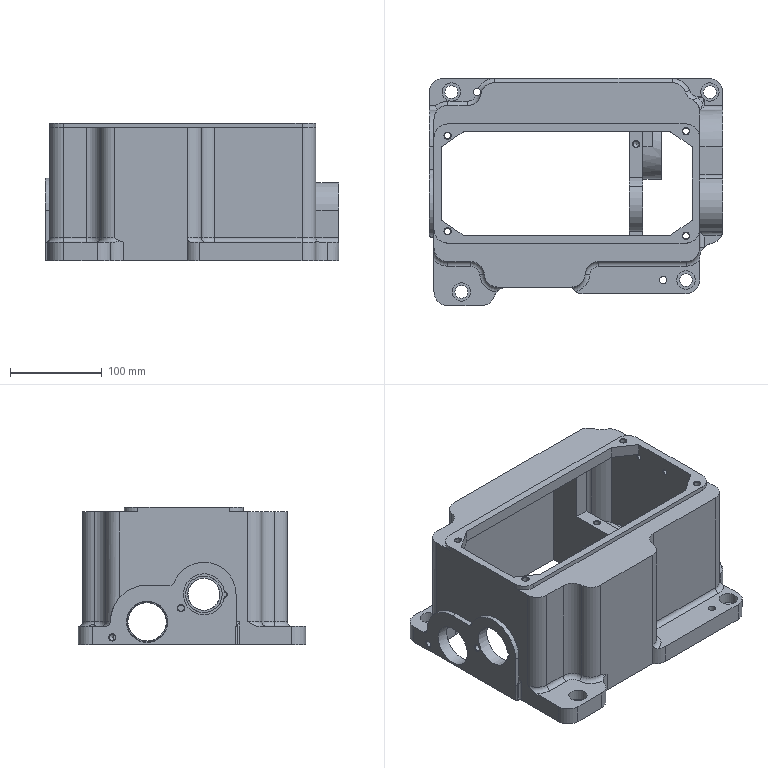Component | NX | LATHE_FEED_BOX | 1 solid | 189 faces | volume 1884837 mm3 | cylinder 88 | plane 64 | cone 24 | torus 11 | spline 2 | commonest cylinder face diameters 30 x26 10 x14 14 x11 6.8 x9 46 x4 20 x4 5 x3 4 x2